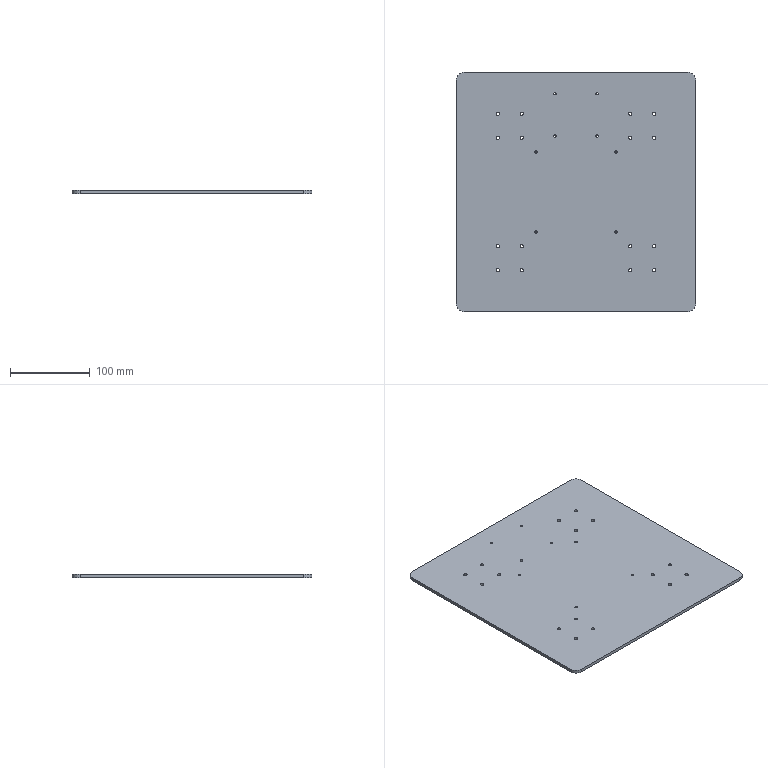Component | SolidWorks | Chassis-1 | 1 solid | 60 faces | box 300 x 300 x 4 mm | volume 358543 mm3 | cylinder 52 | plane 6 | cone 2 | commonest cylinder face diameters 4.2 x32 3 x16 20 x4
build123d program:
from build123d import *

# Parameters (mm, degrees)
SKETCH1_R           = 2.1
BOSS_EXTRUDE1_DEPTH = 4
SKETCH3_R           = 1.5
CUT_EXTRUDE1_DEPTH  = 10
SKETCH4_R           = 1.5
CUT_EXTRUDE2_DEPTH  = 20
CHAMFER1_SIZE       = 0.3


with BuildPart() as part:
    # Sketch1 → Boss-Extrude1 (new body)
    with BuildSketch(Plane.XY):
        with BuildLine():
            Line((-140, -150), (140, -150))
            ThreePointArc((140, -150), (147.071, -147.071), (150, -140))
            Line((150, -140), (150, 140))
            ThreePointArc((150, 140), (147.071, 147.071), (140, 150))
            Line((140, 150), (-140, 150))
            ThreePointArc((-140, 150), (-147.071, 147.071), (-150, 140))
            Line((-150, 140), (-150, -140))
            ThreePointArc((-150, -140), (-147.071, -147.071), (-140, -150))
        make_face()
        with Locations((-98, 98)):
            Circle(SKETCH1_R, mode=Mode.SUBTRACT)
        with Locations(Location((-68, 98, 0), (0, 0, 180))):
            Circle(SKETCH1_R, mode=Mode.SUBTRACT)
        with Locations((-68, 68)):
            Circle(SKETCH1_R, mode=Mode.SUBTRACT)
        with Locations(Location((-98, 68, 0), (0, 0, 180))):
            Circle(SKETCH1_R, mode=Mode.SUBTRACT)
        with Locations(Location((68, 68, 0), (0, 0, 180))):
            Circle(SKETCH1_R, mode=Mode.SUBTRACT)
        with Locations((98, 68)):
            Circle(SKETCH1_R, mode=Mode.SUBTRACT)
        with Locations((68, 98)):
            Circle(SKETCH1_R, mode=Mode.SUBTRACT)
        with Locations(Location((98, 98, 0), (0, 0, 180))):
            Circle(SKETCH1_R, mode=Mode.SUBTRACT)
        with Locations((98, -98)):
            Circle(SKETCH1_R, mode=Mode.SUBTRACT)
        with Locations(Location((68, -98, 0), (0, 0, 180))):
            Circle(SKETCH1_R, mode=Mode.SUBTRACT)
        with Locations((68, -68)):
            Circle(SKETCH1_R, mode=Mode.SUBTRACT)
        with Locations(Location((98, -68, 0), (0, 0, 180))):
            Circle(SKETCH1_R, mode=Mode.SUBTRACT)
        with Locations(Location((-68, -68, 0), (0, 0, 180))):
            Circle(SKETCH1_R, mode=Mode.SUBTRACT)
        with Locations((-98, -68)):
            Circle(SKETCH1_R, mode=Mode.SUBTRACT)
        with Locations((-68, -98)):
            Circle(SKETCH1_R, mode=Mode.SUBTRACT)
        with Locations(Location((-98, -98, 0), (0, 0, 180))):
            Circle(SKETCH1_R, mode=Mode.SUBTRACT)
    extrude(amount=BOSS_EXTRUDE1_DEPTH)

    # Sketch3 → Cut-Extrude1 (cut)
    with BuildSketch(Plane.XY.offset(4)):
        with Locations((-50, 50)):
            Circle(SKETCH3_R)
        with Locations((50, 50)):
            Circle(SKETCH3_R)
        with Locations((50, -50)):
            Circle(SKETCH3_R)
        with Locations((-50, -50)):
            Circle(SKETCH3_R)
    extrude(amount=-CUT_EXTRUDE1_DEPTH, mode=Mode.SUBTRACT)

    # Sketch4 → Cut-Extrude2 (cut)
    with BuildSketch(Plane.XY.offset(4)):
        with Locations((-26.5, 123)):
            Circle(SKETCH4_R)
        with Locations((26.5, 123)):
            Circle(SKETCH4_R)
        with Locations((26.5, 70)):
            Circle(SKETCH4_R)
        with Locations((-26.5, 70)):
            Circle(SKETCH4_R)
    extrude(amount=-CUT_EXTRUDE2_DEPTH, mode=Mode.SUBTRACT)

    # Chamfer1
    chamfer1_edges = [part.edges().sort_by_distance(p)[0] for p in [
        (-51.5, -50, 0),
    ]]
    chamfer(chamfer1_edges, length=CHAMFER1_SIZE)


solid = part.part